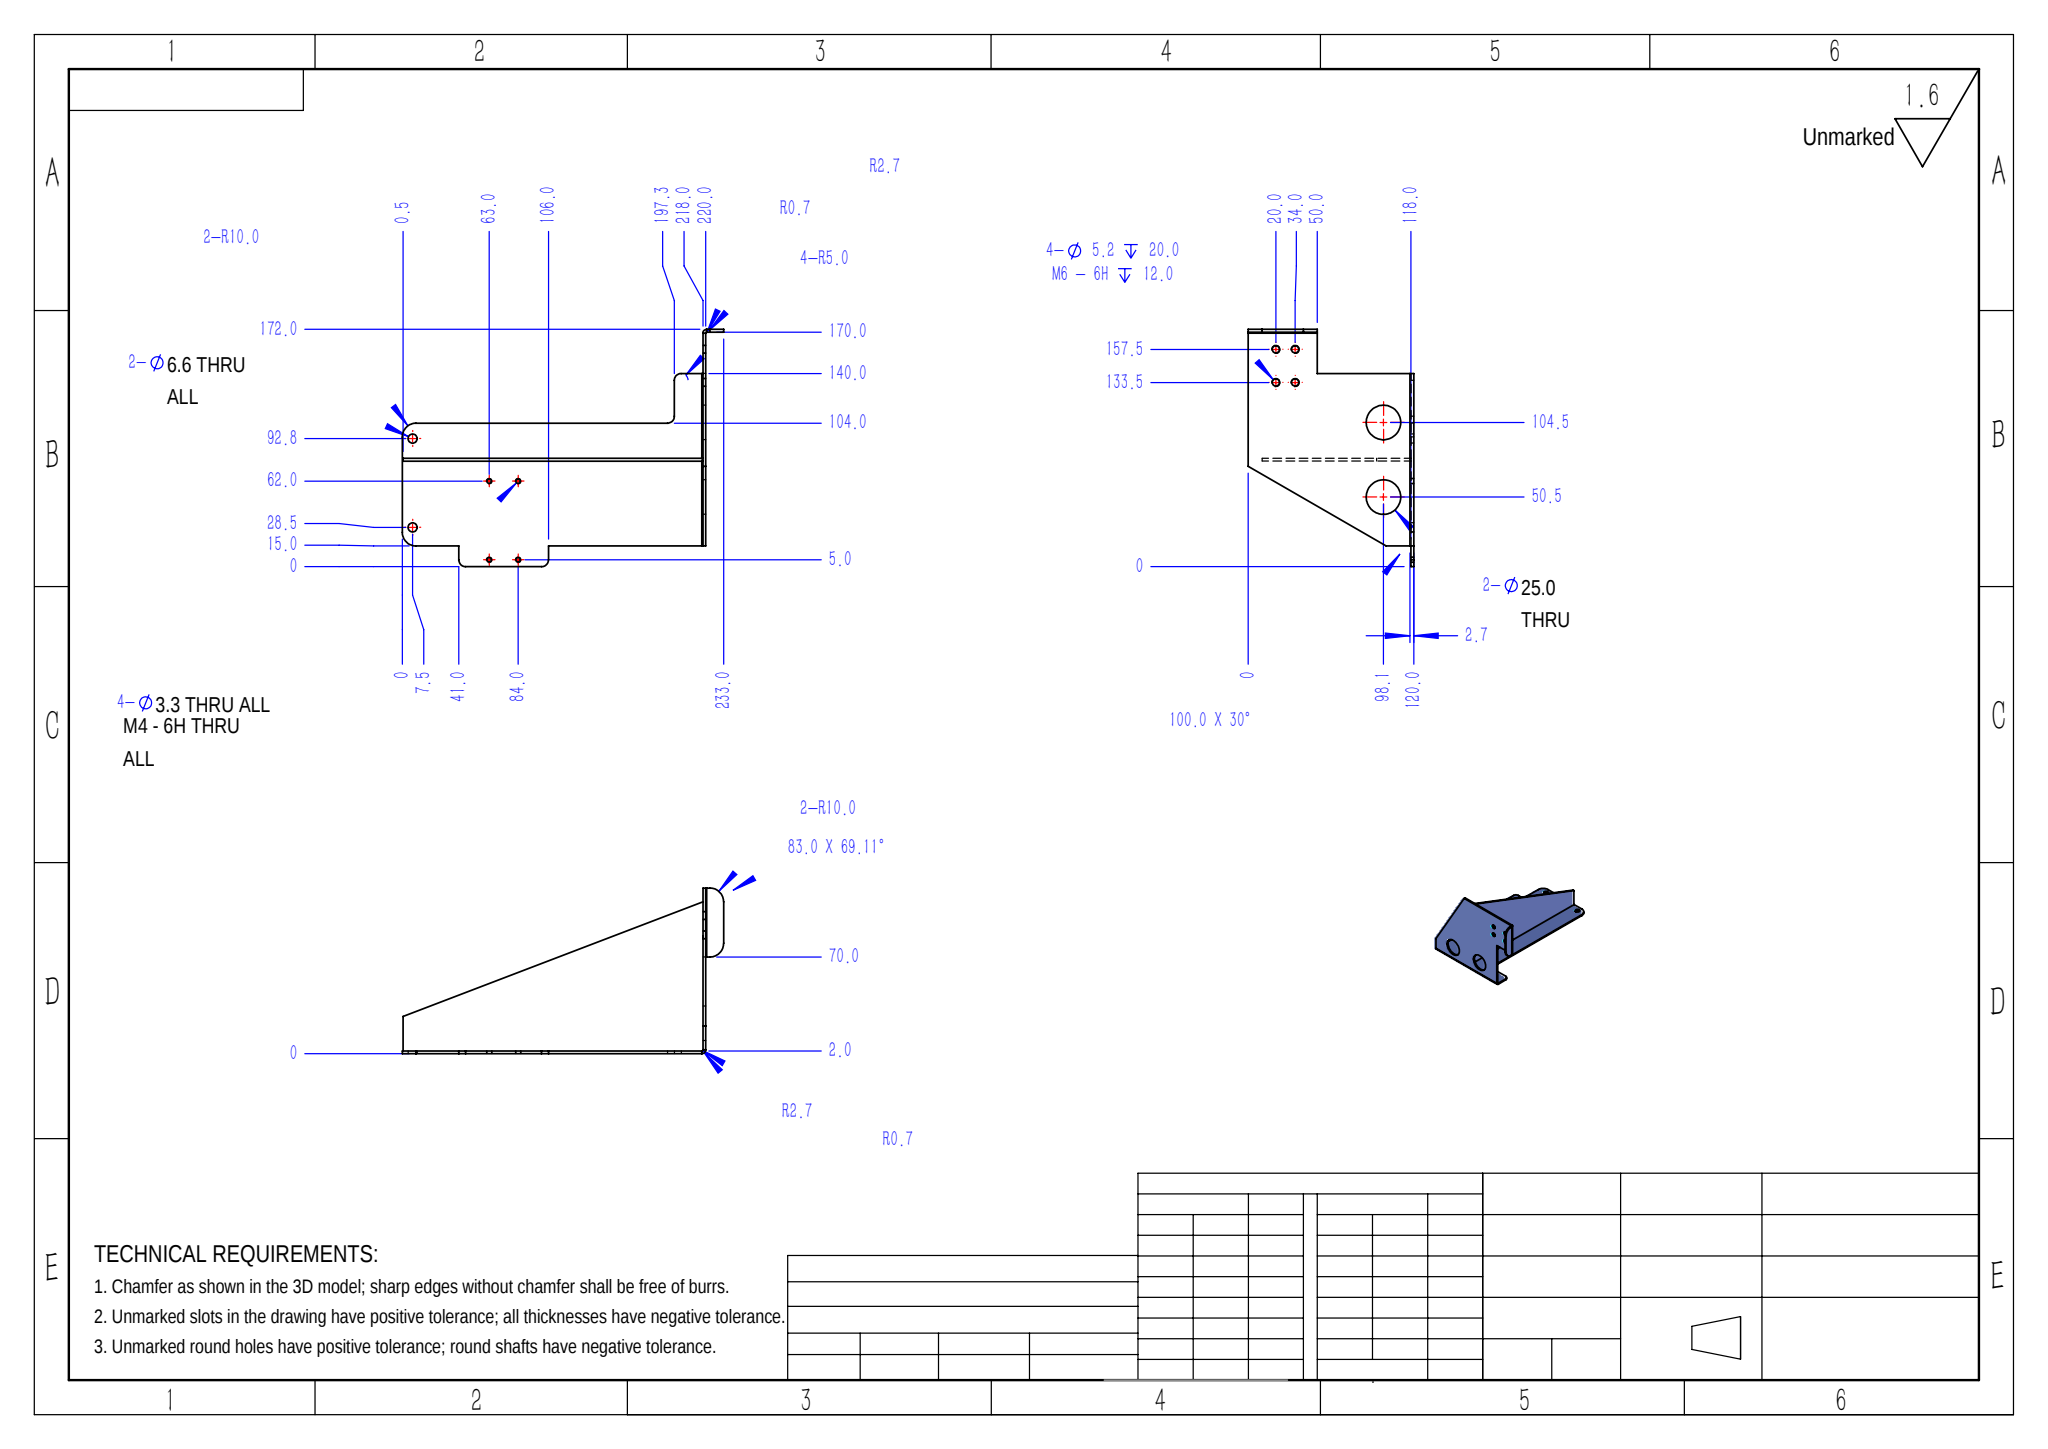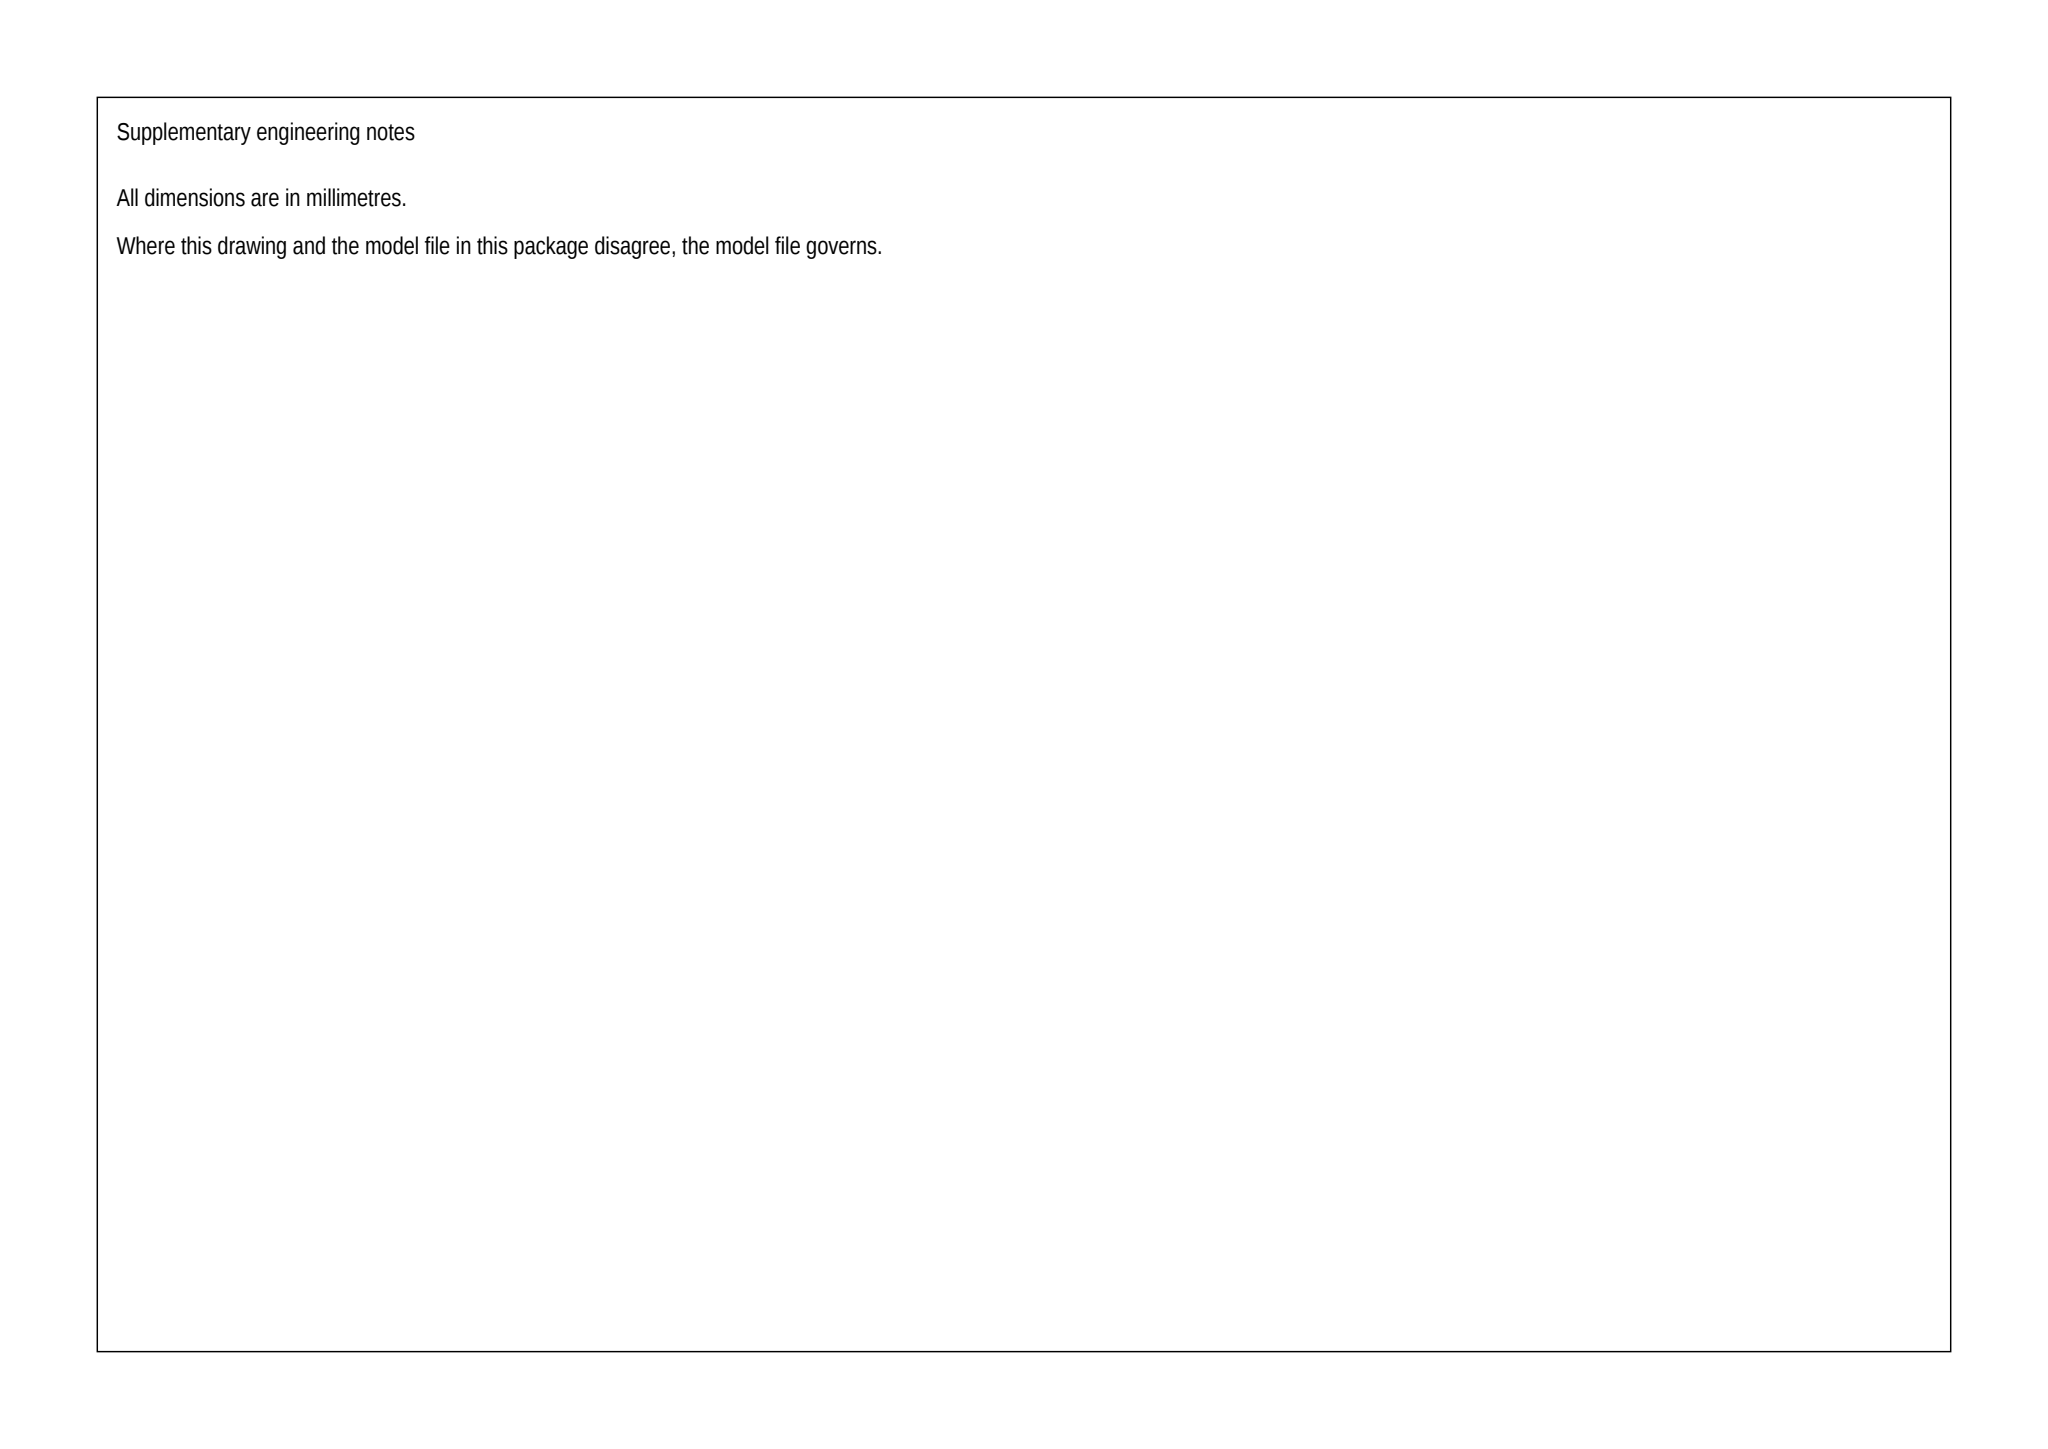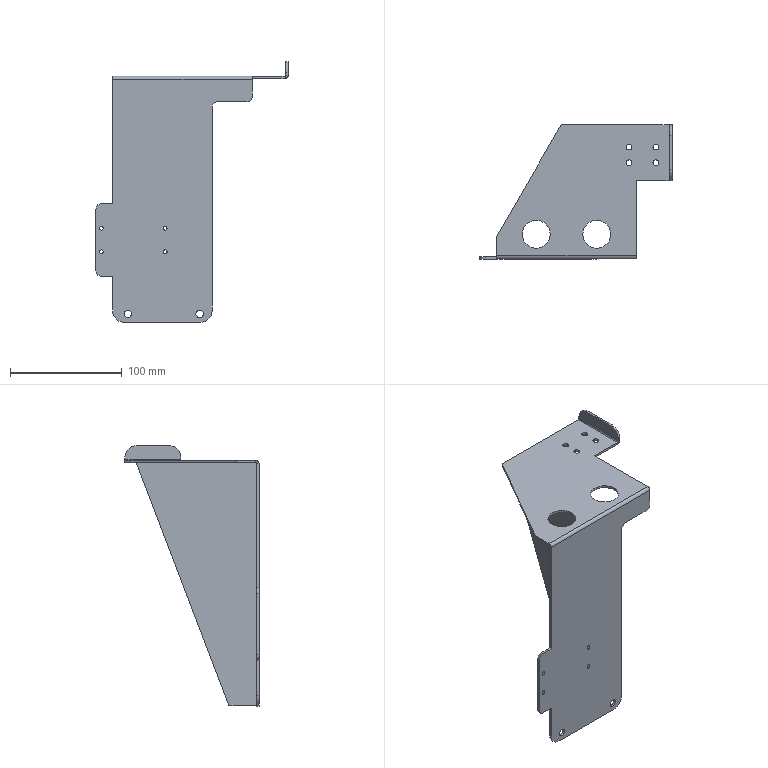Part | SolidWorks | mm | 1 solid | 68 faces | box 172 x 120 x 233 mm | volume 97108 mm3 | cylinder 37 | plane 31 | commonest cylinder face diameters 3.3 x8 5.2 x8 25 x4 6.6 x4 20 x4 10 x4 1.473 x3 5.473 x2